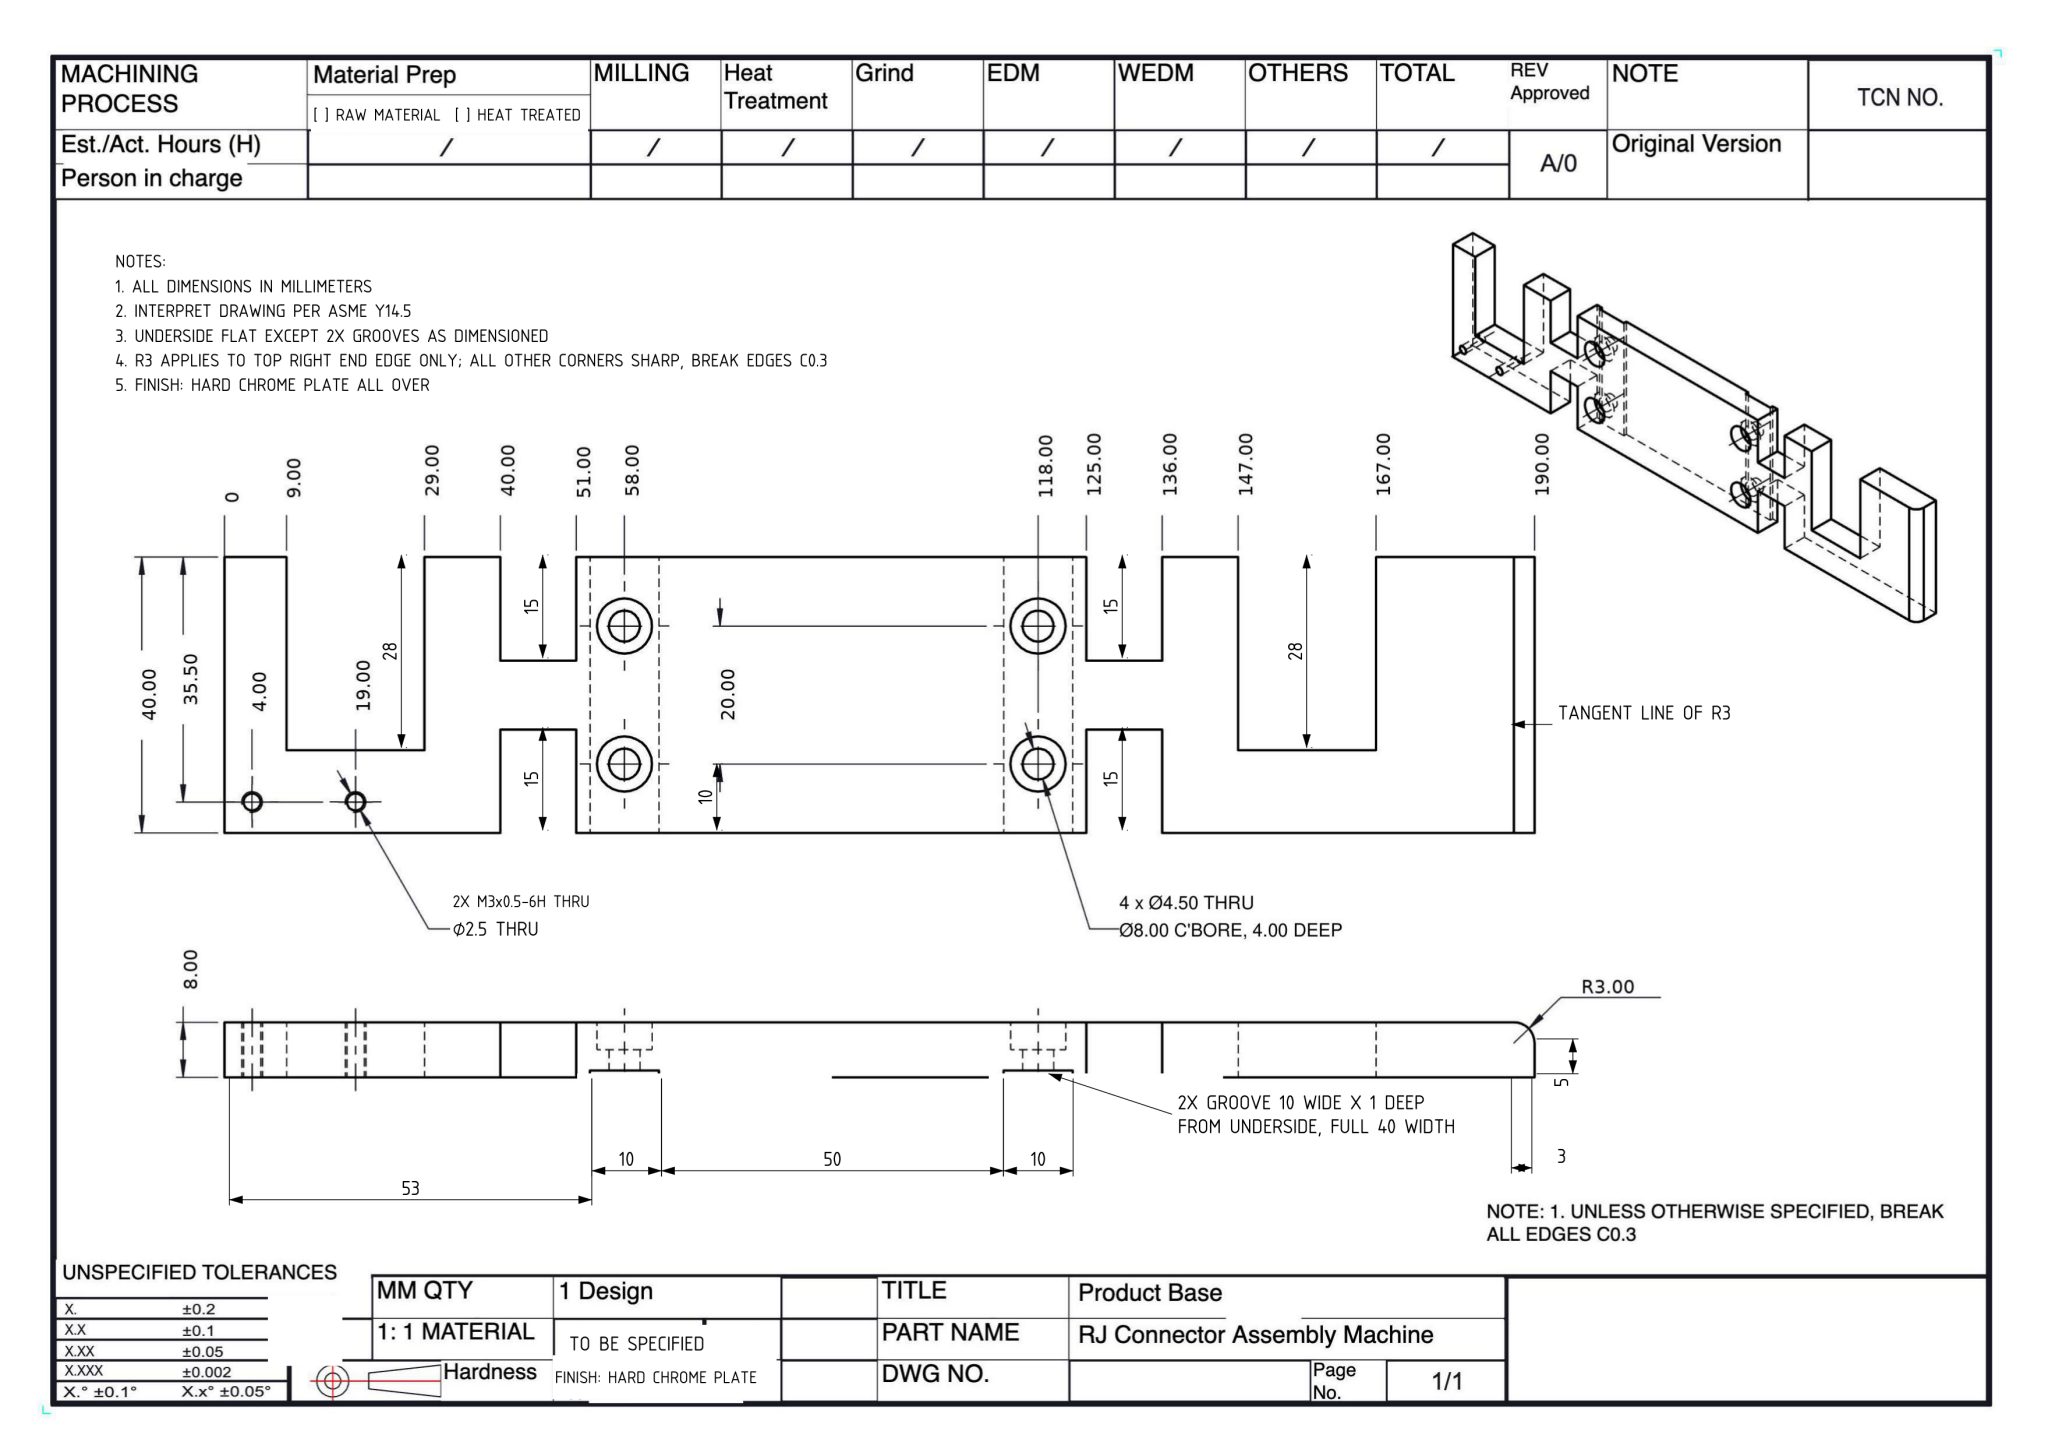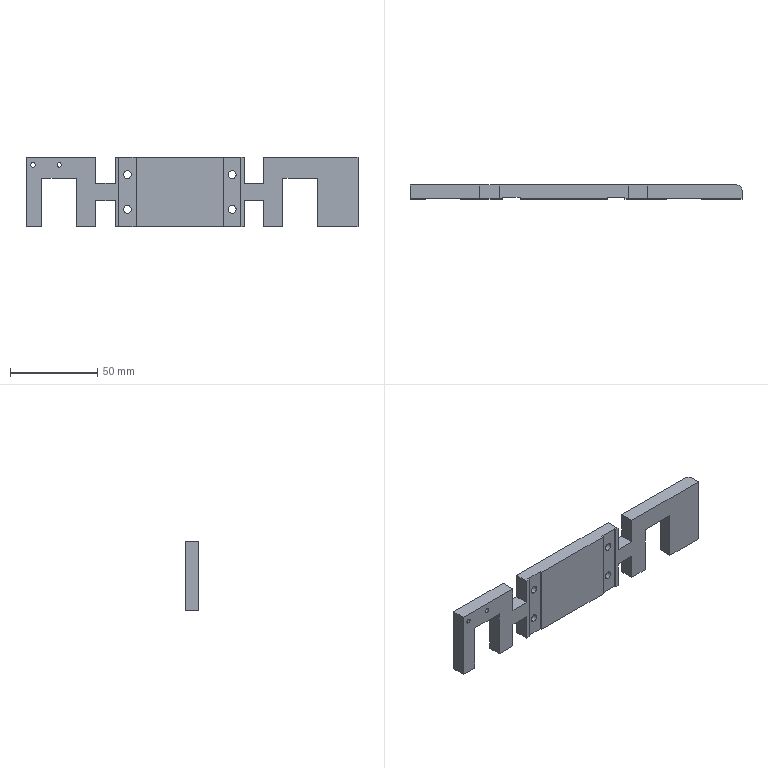Part | NX | mm | 1 solid | 63 faces | box 190 x 8 x 40 mm | volume 44609 mm3 | plane 42 | cylinder 21 | commonest cylinder face diameters 8 x8 4.5 x8 2.5 x4 6 x1